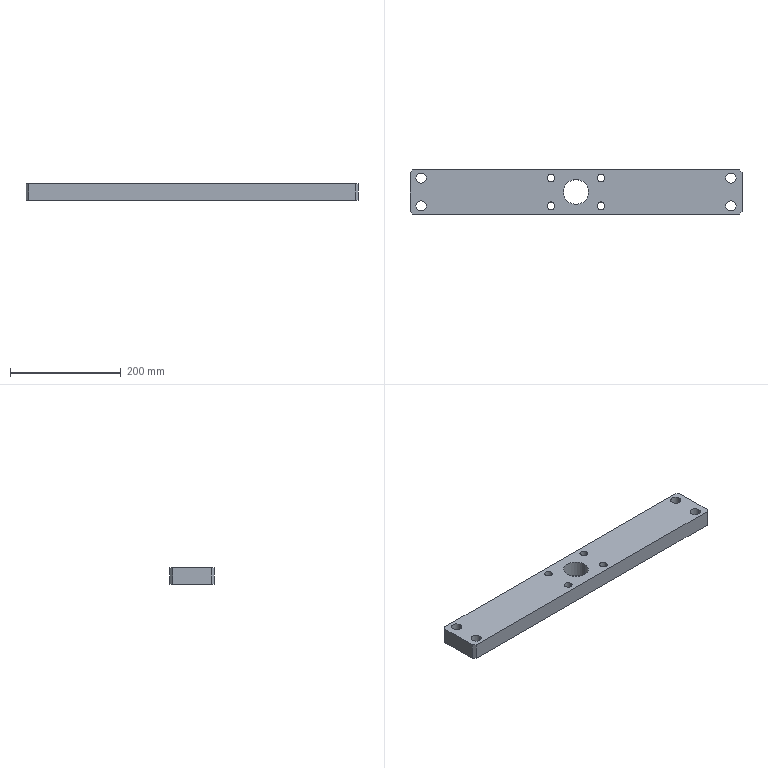Component | SolidWorks | YC1-250-03-01SliderAssembly-1_YC1-250-03-23HydraulicCylinderPressurePlate-1 | 1 solid | 28 faces | box 600 x 80 x 30 mm | volume 1340058 mm3 | cylinder 18 | plane 10 | commonest cylinder face diameters 18.5 x8 14 x8 45 x2 | material Plain Carbon Steel
STEP:
#1=COLOUR_RGB('',0.7922,0.8196,0.9333);
#2=FILL_AREA_STYLE_COLOUR('',#1);
#3=FILL_AREA_STYLE('',(#2));
#4=SURFACE_STYLE_FILL_AREA(#3);
#5=SURFACE_SIDE_STYLE('',(#4));
#6=SURFACE_STYLE_USAGE(.BOTH.,#5);
#7=PRESENTATION_STYLE_ASSIGNMENT((#6));
#8=CARTESIAN_POINT('',(11.388,79.214,-8.465));
#9=VERTEX_POINT('',#8);
#10=CARTESIAN_POINT('',(10.659,79.214,-8.465));
#11=VERTEX_POINT('',#10);
#12=CARTESIAN_POINT('',(11.024,79.214,-8.465));
#13=DIRECTION('',(0.,0.,-1.));
#14=DIRECTION('',(-1.,0.,0.));
#15=AXIS2_PLACEMENT_3D('',#12,#13,#14);
#16=CIRCLE('',#15,0.3642);
#17=EDGE_CURVE('',#9,#11,#16,.T.);
#18=ORIENTED_EDGE('',*,*,#17,.F.);
#19=CARTESIAN_POINT('',(11.388,79.214,-9.646));
#20=VERTEX_POINT('',#19);
#21=CARTESIAN_POINT('',(11.388,79.214,-9.646));
#22=DIRECTION('',(0.,0.,-1.));
#23=VECTOR('',#22,39.37);
#24=LINE('',#21,#23);
#25=EDGE_CURVE('',#9,#20,#24,.T.);
#26=ORIENTED_EDGE('',*,*,#25,.T.);
#27=CARTESIAN_POINT('',(10.659,79.214,-9.646));
#28=VERTEX_POINT('',#27);
#29=CARTESIAN_POINT('',(11.024,79.214,-9.646));
#30=DIRECTION('',(0.,0.,-1.));
#31=DIRECTION('',(-1.,0.,0.));
#32=AXIS2_PLACEMENT_3D('',#29,#30,#31);
#33=CIRCLE('',#32,0.3642);
#34=EDGE_CURVE('',#20,#28,#33,.T.);
#35=ORIENTED_EDGE('',*,*,#34,.T.);
#36=CARTESIAN_POINT('',(10.659,79.214,-9.646));
#37=DIRECTION('',(0.,0.,-1.));
#38=VECTOR('',#37,39.37);
#39=LINE('',#36,#38);
#40=EDGE_CURVE('',#11,#28,#39,.T.);
#41=ORIENTED_EDGE('',*,*,#40,.F.);
#42=EDGE_LOOP('',(#18,#26,#35,#41));
#43=FACE_OUTER_BOUND('',#42,.T.);
#44=CARTESIAN_POINT('',(11.024,79.214,-9.646));
#45=DIRECTION('',(0.,0.,-1.));
#46=DIRECTION('',(-1.,0.,0.));
#47=AXIS2_PLACEMENT_3D('',#44,#45,#46);
#48=CYLINDRICAL_SURFACE('',#47,0.3642);
#49=ADVANCED_FACE('',(#43),#48,.F.);
#50=CARTESIAN_POINT('',(11.388,77.246,-8.465));
#51=VERTEX_POINT('',#50);
#52=CARTESIAN_POINT('',(10.659,77.246,-8.465));
#53=VERTEX_POINT('',#52);
#54=CARTESIAN_POINT('',(11.024,77.246,-8.465));
#55=DIRECTION('',(0.,0.,-1.));
#56=DIRECTION('',(-1.,0.,0.));
#57=AXIS2_PLACEMENT_3D('',#54,#55,#56);
#58=CIRCLE('',#57,0.3642);
#59=EDGE_CURVE('',#51,#53,#58,.T.);
#60=ORIENTED_EDGE('',*,*,#59,.F.);
#61=CARTESIAN_POINT('',(11.388,77.246,-9.646));
#62=VERTEX_POINT('',#61);
#63=CARTESIAN_POINT('',(11.388,77.246,-9.646));
#64=DIRECTION('',(0.,0.,-1.));
#65=VECTOR('',#64,39.37);
#66=LINE('',#63,#65);
#67=EDGE_CURVE('',#51,#62,#66,.T.);
#68=ORIENTED_EDGE('',*,*,#67,.T.);
#69=CARTESIAN_POINT('',(10.659,77.246,-9.646));
#70=VERTEX_POINT('',#69);
#71=CARTESIAN_POINT('',(11.024,77.246,-9.646));
#72=DIRECTION('',(0.,0.,-1.));
#73=DIRECTION('',(-1.,0.,0.));
#74=AXIS2_PLACEMENT_3D('',#71,#72,#73);
#75=CIRCLE('',#74,0.3642);
#76=EDGE_CURVE('',#62,#70,#75,.T.);
#77=ORIENTED_EDGE('',*,*,#76,.T.);
#78=CARTESIAN_POINT('',(10.659,77.246,-9.646));
#79=DIRECTION('',(0.,0.,-1.));
#80=VECTOR('',#79,39.37);
#81=LINE('',#78,#80);
#82=EDGE_CURVE('',#53,#70,#81,.T.);
#83=ORIENTED_EDGE('',*,*,#82,.F.);
#84=EDGE_LOOP('',(#60,#68,#77,#83));
#85=FACE_OUTER_BOUND('',#84,.T.);
#86=CARTESIAN_POINT('',(11.024,77.246,-9.646));
#87=DIRECTION('',(0.,0.,-1.));
#88=DIRECTION('',(-1.,0.,0.));
#89=AXIS2_PLACEMENT_3D('',#86,#87,#88);
#90=CYLINDRICAL_SURFACE('',#89,0.3642);
#91=ADVANCED_FACE('',(#85),#90,.F.);
#92=CARTESIAN_POINT('',(-10.659,77.246,-8.465));
#93=VERTEX_POINT('',#92);
#94=CARTESIAN_POINT('',(-11.388,77.246,-8.465));
#95=VERTEX_POINT('',#94);
#96=CARTESIAN_POINT('',(-11.024,77.246,-8.465));
#97=DIRECTION('',(0.,0.,-1.));
#98=DIRECTION('',(-1.,0.,0.));
#99=AXIS2_PLACEMENT_3D('',#96,#97,#98);
#100=CIRCLE('',#99,0.3642);
#101=EDGE_CURVE('',#93,#95,#100,.T.);
#102=ORIENTED_EDGE('',*,*,#101,.F.);
#103=CARTESIAN_POINT('',(-10.659,77.246,-9.646));
#104=VERTEX_POINT('',#103);
#105=CARTESIAN_POINT('',(-10.659,77.246,-9.646));
#106=DIRECTION('',(0.,0.,-1.));
#107=VECTOR('',#106,39.37);
#108=LINE('',#105,#107);
#109=EDGE_CURVE('',#93,#104,#108,.T.);
#110=ORIENTED_EDGE('',*,*,#109,.T.);
#111=CARTESIAN_POINT('',(-11.388,77.246,-9.646));
#112=VERTEX_POINT('',#111);
#113=CARTESIAN_POINT('',(-11.024,77.246,-9.646));
#114=DIRECTION('',(0.,0.,-1.));
#115=DIRECTION('',(-1.,0.,0.));
#116=AXIS2_PLACEMENT_3D('',#113,#114,#115);
#117=CIRCLE('',#116,0.3642);
#118=EDGE_CURVE('',#104,#112,#117,.T.);
#119=ORIENTED_EDGE('',*,*,#118,.T.);
#120=CARTESIAN_POINT('',(-11.388,77.246,-9.646));
#121=DIRECTION('',(0.,0.,-1.));
#122=VECTOR('',#121,39.37);
#123=LINE('',#120,#122);
#124=EDGE_CURVE('',#95,#112,#123,.T.);
#125=ORIENTED_EDGE('',*,*,#124,.F.);
#126=EDGE_LOOP('',(#102,#110,#119,#125));
#127=FACE_OUTER_BOUND('',#126,.T.);
#128=CARTESIAN_POINT('',(-11.024,77.246,-9.646));
#129=DIRECTION('',(0.,0.,-1.));
#130=DIRECTION('',(-1.,0.,0.));
#131=AXIS2_PLACEMENT_3D('',#128,#129,#130);
#132=CYLINDRICAL_SURFACE('',#131,0.3642);
#133=ADVANCED_FACE('',(#127),#132,.F.);
#134=CARTESIAN_POINT('',(-10.659,79.214,-8.465));
#135=VERTEX_POINT('',#134);
#136=CARTESIAN_POINT('',(-11.388,79.214,-8.465));
#137=VERTEX_POINT('',#136);
#138=CARTESIAN_POINT('',(-11.024,79.214,-8.465));
#139=DIRECTION('',(0.,0.,-1.));
#140=DIRECTION('',(-1.,0.,0.));
#141=AXIS2_PLACEMENT_3D('',#138,#139,#140);
#142=CIRCLE('',#141,0.3642);
#143=EDGE_CURVE('',#135,#137,#142,.T.);
#144=ORIENTED_EDGE('',*,*,#143,.F.);
#145=CARTESIAN_POINT('',(-10.659,79.214,-9.646));
#146=VERTEX_POINT('',#145);
#147=CARTESIAN_POINT('',(-10.659,79.214,-9.646));
#148=DIRECTION('',(0.,0.,-1.));
#149=VECTOR('',#148,39.37);
#150=LINE('',#147,#149);
#151=EDGE_CURVE('',#135,#146,#150,.T.);
#152=ORIENTED_EDGE('',*,*,#151,.T.);
#153=CARTESIAN_POINT('',(-11.388,79.214,-9.646));
#154=VERTEX_POINT('',#153);
#155=CARTESIAN_POINT('',(-11.024,79.214,-9.646));
#156=DIRECTION('',(0.,0.,-1.));
#157=DIRECTION('',(-1.,0.,0.));
#158=AXIS2_PLACEMENT_3D('',#155,#156,#157);
#159=CIRCLE('',#158,0.3642);
#160=EDGE_CURVE('',#146,#154,#159,.T.);
#161=ORIENTED_EDGE('',*,*,#160,.T.);
#162=CARTESIAN_POINT('',(-11.388,79.214,-9.646));
#163=DIRECTION('',(0.,0.,-1.));
#164=VECTOR('',#163,39.37);
#165=LINE('',#162,#164);
#166=EDGE_CURVE('',#137,#154,#165,.T.);
#167=ORIENTED_EDGE('',*,*,#166,.F.);
#168=EDGE_LOOP('',(#144,#152,#161,#167));
#169=FACE_OUTER_BOUND('',#168,.T.);
#170=CARTESIAN_POINT('',(-11.024,79.214,-9.646));
#171=DIRECTION('',(0.,0.,-1.));
#172=DIRECTION('',(-1.,0.,0.));
#173=AXIS2_PLACEMENT_3D('',#170,#171,#172);
#174=CYLINDRICAL_SURFACE('',#173,0.3642);
#175=ADVANCED_FACE('',(#169),#174,.F.);
#176=CARTESIAN_POINT('',(0.8858,78.23,-8.465));
#177=VERTEX_POINT('',#176);
#178=CARTESIAN_POINT('',(-0.8858,78.23,-8.465));
#179=VERTEX_POINT('',#178);
#180=CARTESIAN_POINT('',(0.,78.23,-8.465));
#181=DIRECTION('',(0.,0.,-1.));
#182=DIRECTION('',(-1.,0.,0.));
#183=AXIS2_PLACEMENT_3D('',#180,#181,#182);
#184=CIRCLE('',#183,0.8858);
#185=EDGE_CURVE('',#177,#179,#184,.T.);
#186=ORIENTED_EDGE('',*,*,#185,.F.);
#187=CARTESIAN_POINT('',(0.8858,78.23,-9.646));
#188=VERTEX_POINT('',#187);
#189=CARTESIAN_POINT('',(0.8858,78.23,-9.646));
#190=DIRECTION('',(0.,0.,-1.));
#191=VECTOR('',#190,39.37);
#192=LINE('',#189,#191);
#193=EDGE_CURVE('',#177,#188,#192,.T.);
#194=ORIENTED_EDGE('',*,*,#193,.T.);
#195=CARTESIAN_POINT('',(-0.8858,78.23,-9.646));
#196=VERTEX_POINT('',#195);
#197=CARTESIAN_POINT('',(0.,78.23,-9.646));
#198=DIRECTION('',(0.,0.,-1.));
#199=DIRECTION('',(-1.,0.,0.));
#200=AXIS2_PLACEMENT_3D('',#197,#198,#199);
#201=CIRCLE('',#200,0.8858);
#202=EDGE_CURVE('',#188,#196,#201,.T.);
#203=ORIENTED_EDGE('',*,*,#202,.T.);
#204=CARTESIAN_POINT('',(-0.8858,78.23,-9.646));
#205=DIRECTION('',(0.,0.,-1.));
#206=VECTOR('',#205,39.37);
#207=LINE('',#204,#206);
#208=EDGE_CURVE('',#179,#196,#207,.T.);
#209=ORIENTED_EDGE('',*,*,#208,.F.);
#210=EDGE_LOOP('',(#186,#194,#203,#209));
#211=FACE_OUTER_BOUND('',#210,.T.);
#212=CARTESIAN_POINT('',(0.,78.23,-9.646));
#213=DIRECTION('',(0.,0.,-1.));
#214=DIRECTION('',(-1.,0.,0.));
#215=AXIS2_PLACEMENT_3D('',#212,#213,#214);
#216=CYLINDRICAL_SURFACE('',#215,0.8858);
#217=ADVANCED_FACE('',(#211),#216,.F.);
#218=CARTESIAN_POINT('',(-1.496,77.246,-8.465));
#219=VERTEX_POINT('',#218);
#220=CARTESIAN_POINT('',(-2.047,77.246,-8.465));
#221=VERTEX_POINT('',#220);
#222=CARTESIAN_POINT('',(-1.772,77.246,-8.465));
#223=DIRECTION('',(0.,0.,-1.));
#224=DIRECTION('',(-1.,0.,0.));
#225=AXIS2_PLACEMENT_3D('',#222,#223,#224);
#226=CIRCLE('',#225,0.2756);
#227=EDGE_CURVE('',#219,#221,#226,.T.);
#228=ORIENTED_EDGE('',*,*,#227,.F.);
#229=CARTESIAN_POINT('',(-1.496,77.246,-9.646));
#230=VERTEX_POINT('',#229);
#231=CARTESIAN_POINT('',(-1.496,77.246,-9.646));
#232=DIRECTION('',(0.,0.,-1.));
#233=VECTOR('',#232,39.37);
#234=LINE('',#231,#233);
#235=EDGE_CURVE('',#219,#230,#234,.T.);
#236=ORIENTED_EDGE('',*,*,#235,.T.);
#237=CARTESIAN_POINT('',(-2.047,77.246,-9.646));
#238=VERTEX_POINT('',#237);
#239=CARTESIAN_POINT('',(-1.772,77.246,-9.646));
#240=DIRECTION('',(0.,0.,-1.));
#241=DIRECTION('',(-1.,0.,0.));
#242=AXIS2_PLACEMENT_3D('',#239,#240,#241);
#243=CIRCLE('',#242,0.2756);
#244=EDGE_CURVE('',#230,#238,#243,.T.);
#245=ORIENTED_EDGE('',*,*,#244,.T.);
#246=CARTESIAN_POINT('',(-2.047,77.246,-9.646));
#247=DIRECTION('',(0.,0.,-1.));
#248=VECTOR('',#247,39.37);
#249=LINE('',#246,#248);
#250=EDGE_CURVE('',#221,#238,#249,.T.);
#251=ORIENTED_EDGE('',*,*,#250,.F.);
#252=EDGE_LOOP('',(#228,#236,#245,#251));
#253=FACE_OUTER_BOUND('',#252,.T.);
#254=CARTESIAN_POINT('',(-1.772,77.246,-9.646));
#255=DIRECTION('',(0.,0.,-1.));
#256=DIRECTION('',(-1.,0.,0.));
#257=AXIS2_PLACEMENT_3D('',#254,#255,#256);
#258=CYLINDRICAL_SURFACE('',#257,0.2756);
#259=ADVANCED_FACE('',(#253),#258,.F.);
#260=CARTESIAN_POINT('',(2.047,77.246,-8.465));
#261=VERTEX_POINT('',#260);
#262=CARTESIAN_POINT('',(1.496,77.246,-8.465));
#263=VERTEX_POINT('',#262);
#264=CARTESIAN_POINT('',(1.772,77.246,-8.465));
#265=DIRECTION('',(0.,0.,-1.));
#266=DIRECTION('',(-1.,0.,0.));
#267=AXIS2_PLACEMENT_3D('',#264,#265,#266);
#268=CIRCLE('',#267,0.2756);
#269=EDGE_CURVE('',#261,#263,#268,.T.);
#270=ORIENTED_EDGE('',*,*,#269,.F.);
#271=CARTESIAN_POINT('',(2.047,77.246,-9.646));
#272=VERTEX_POINT('',#271);
#273=CARTESIAN_POINT('',(2.047,77.246,-9.646));
#274=DIRECTION('',(0.,0.,-1.));
#275=VECTOR('',#274,39.37);
#276=LINE('',#273,#275);
#277=EDGE_CURVE('',#261,#272,#276,.T.);
#278=ORIENTED_EDGE('',*,*,#277,.T.);
#279=CARTESIAN_POINT('',(1.496,77.246,-9.646));
#280=VERTEX_POINT('',#279);
#281=CARTESIAN_POINT('',(1.772,77.246,-9.646));
#282=DIRECTION('',(0.,0.,-1.));
#283=DIRECTION('',(-1.,0.,0.));
#284=AXIS2_PLACEMENT_3D('',#281,#282,#283);
#285=CIRCLE('',#284,0.2756);
#286=EDGE_CURVE('',#272,#280,#285,.T.);
#287=ORIENTED_EDGE('',*,*,#286,.T.);
#288=CARTESIAN_POINT('',(1.496,77.246,-9.646));
#289=DIRECTION('',(0.,0.,-1.));
#290=VECTOR('',#289,39.37);
#291=LINE('',#288,#290);
#292=EDGE_CURVE('',#263,#280,#291,.T.);
#293=ORIENTED_EDGE('',*,*,#292,.F.);
#294=EDGE_LOOP('',(#270,#278,#287,#293));
#295=FACE_OUTER_BOUND('',#294,.T.);
#296=CARTESIAN_POINT('',(1.772,77.246,-9.646));
#297=DIRECTION('',(0.,0.,-1.));
#298=DIRECTION('',(-1.,0.,0.));
#299=AXIS2_PLACEMENT_3D('',#296,#297,#298);
#300=CYLINDRICAL_SURFACE('',#299,0.2756);
#301=ADVANCED_FACE('',(#295),#300,.F.);
#302=CARTESIAN_POINT('',(2.047,79.214,-8.465));
#303=VERTEX_POINT('',#302);
#304=CARTESIAN_POINT('',(1.496,79.214,-8.465));
#305=VERTEX_POINT('',#304);
#306=CARTESIAN_POINT('',(1.772,79.214,-8.465));
#307=DIRECTION('',(0.,0.,-1.));
#308=DIRECTION('',(-1.,0.,0.));
#309=AXIS2_PLACEMENT_3D('',#306,#307,#308);
#310=CIRCLE('',#309,0.2756);
#311=EDGE_CURVE('',#303,#305,#310,.T.);
#312=ORIENTED_EDGE('',*,*,#311,.F.);
#313=CARTESIAN_POINT('',(2.047,79.214,-9.646));
#314=VERTEX_POINT('',#313);
#315=CARTESIAN_POINT('',(2.047,79.214,-9.646));
#316=DIRECTION('',(0.,0.,-1.));
#317=VECTOR('',#316,39.37);
#318=LINE('',#315,#317);
#319=EDGE_CURVE('',#303,#314,#318,.T.);
#320=ORIENTED_EDGE('',*,*,#319,.T.);
#321=CARTESIAN_POINT('',(1.496,79.214,-9.646));
#322=VERTEX_POINT('',#321);
#323=CARTESIAN_POINT('',(1.772,79.214,-9.646));
#324=DIRECTION('',(0.,0.,-1.));
#325=DIRECTION('',(-1.,0.,0.));
#326=AXIS2_PLACEMENT_3D('',#323,#324,#325);
#327=CIRCLE('',#326,0.2756);
#328=EDGE_CURVE('',#314,#322,#327,.T.);
#329=ORIENTED_EDGE('',*,*,#328,.T.);
#330=CARTESIAN_POINT('',(1.496,79.214,-9.646));
#331=DIRECTION('',(0.,0.,-1.));
#332=VECTOR('',#331,39.37);
#333=LINE('',#330,#332);
#334=EDGE_CURVE('',#305,#322,#333,.T.);
#335=ORIENTED_EDGE('',*,*,#334,.F.);
#336=EDGE_LOOP('',(#312,#320,#329,#335));
#337=FACE_OUTER_BOUND('',#336,.T.);
#338=CARTESIAN_POINT('',(1.772,79.214,-9.646));
#339=DIRECTION('',(0.,0.,-1.));
#340=DIRECTION('',(-1.,0.,0.));
#341=AXIS2_PLACEMENT_3D('',#338,#339,#340);
#342=CYLINDRICAL_SURFACE('',#341,0.2756);
#343=ADVANCED_FACE('',(#337),#342,.F.);
#344=CARTESIAN_POINT('',(-1.496,79.214,-8.465));
#345=VERTEX_POINT('',#344);
#346=CARTESIAN_POINT('',(-2.047,79.214,-8.465));
#347=VERTEX_POINT('',#346);
#348=CARTESIAN_POINT('',(-1.772,79.214,-8.465));
#349=DIRECTION('',(0.,0.,-1.));
#350=DIRECTION('',(-1.,0.,0.));
#351=AXIS2_PLACEMENT_3D('',#348,#349,#350);
#352=CIRCLE('',#351,0.2756);
#353=EDGE_CURVE('',#345,#347,#352,.T.);
#354=ORIENTED_EDGE('',*,*,#353,.F.);
#355=CARTESIAN_POINT('',(-1.496,79.214,-9.646));
#356=VERTEX_POINT('',#355);
#357=CARTESIAN_POINT('',(-1.496,79.214,-9.646));
#358=DIRECTION('',(0.,0.,-1.));
#359=VECTOR('',#358,39.37);
#360=LINE('',#357,#359);
#361=EDGE_CURVE('',#345,#356,#360,.T.);
#362=ORIENTED_EDGE('',*,*,#361,.T.);
#363=CARTESIAN_POINT('',(-2.047,79.214,-9.646));
#364=VERTEX_POINT('',#363);
#365=CARTESIAN_POINT('',(-1.772,79.214,-9.646));
#366=DIRECTION('',(0.,0.,-1.));
#367=DIRECTION('',(-1.,0.,0.));
#368=AXIS2_PLACEMENT_3D('',#365,#366,#367);
#369=CIRCLE('',#368,0.2756);
#370=EDGE_CURVE('',#356,#364,#369,.T.);
#371=ORIENTED_EDGE('',*,*,#370,.T.);
#372=CARTESIAN_POINT('',(-2.047,79.214,-9.646));
#373=DIRECTION('',(0.,0.,-1.));
#374=VECTOR('',#373,39.37);
#375=LINE('',#372,#374);
#376=EDGE_CURVE('',#347,#364,#375,.T.);
#377=ORIENTED_EDGE('',*,*,#376,.F.);
#378=EDGE_LOOP('',(#354,#362,#371,#377));
#379=FACE_OUTER_BOUND('',#378,.T.);
#380=CARTESIAN_POINT('',(-1.772,79.214,-9.646));
#381=DIRECTION('',(0.,0.,-1.));
#382=DIRECTION('',(-1.,0.,0.));
#383=AXIS2_PLACEMENT_3D('',#380,#381,#382);
#384=CYLINDRICAL_SURFACE('',#383,0.2756);
#385=ADVANCED_FACE('',(#379),#384,.F.);
#386=CARTESIAN_POINT('',(11.614,76.655,-9.646));
#387=VERTEX_POINT('',#386);
#388=CARTESIAN_POINT('',(11.811,76.852,-9.646));
#389=VERTEX_POINT('',#388);
#390=CARTESIAN_POINT('',(11.614,76.655,-9.646));
#391=DIRECTION('',(0.7071,0.7071,0.));
#392=VECTOR('',#391,39.37);
#393=LINE('',#390,#392);
#394=EDGE_CURVE('',#387,#389,#393,.T.);
#395=ORIENTED_EDGE('',*,*,#394,.F.);
#396=CARTESIAN_POINT('',(-11.614,76.655,-9.646));
#397=VERTEX_POINT('',#396);
#398=CARTESIAN_POINT('',(-11.811,76.655,-9.646));
#399=DIRECTION('',(1.,0.,0.));
#400=VECTOR('',#399,39.37);
#401=LINE('',#398,#400);
#402=EDGE_CURVE('',#397,#387,#401,.T.);
#403=ORIENTED_EDGE('',*,*,#402,.F.);
#404=CARTESIAN_POINT('',(-11.811,76.852,-9.646));
#405=VERTEX_POINT('',#404);
#406=CARTESIAN_POINT('',(-11.811,76.852,-9.646));
#407=DIRECTION('',(0.7071,-0.7071,0.));
#408=VECTOR('',#407,39.37);
#409=LINE('',#406,#408);
#410=EDGE_CURVE('',#405,#397,#409,.T.);
#411=ORIENTED_EDGE('',*,*,#410,.F.);
#412=CARTESIAN_POINT('',(-11.811,79.608,-9.646));
#413=VERTEX_POINT('',#412);
#414=CARTESIAN_POINT('',(-11.811,76.655,-9.646));
#415=DIRECTION('',(0.,-1.,0.));
#416=VECTOR('',#415,39.37);
#417=LINE('',#414,#416);
#418=EDGE_CURVE('',#413,#405,#417,.T.);
#419=ORIENTED_EDGE('',*,*,#418,.F.);
#420=CARTESIAN_POINT('',(-11.614,79.805,-9.646));
#421=VERTEX_POINT('',#420);
#422=CARTESIAN_POINT('',(-11.614,79.805,-9.646));
#423=DIRECTION('',(-0.7071,-0.7071,0.));
#424=VECTOR('',#423,39.37);
#425=LINE('',#422,#424);
#426=EDGE_CURVE('',#421,#413,#425,.T.);
#427=ORIENTED_EDGE('',*,*,#426,.F.);
#428=CARTESIAN_POINT('',(11.614,79.805,-9.646));
#429=VERTEX_POINT('',#428);
#430=CARTESIAN_POINT('',(-11.811,79.805,-9.646));
#431=DIRECTION('',(-1.,0.,0.));
#432=VECTOR('',#431,39.37);
#433=LINE('',#430,#432);
#434=EDGE_CURVE('',#429,#421,#433,.T.);
#435=ORIENTED_EDGE('',*,*,#434,.F.);
#436=CARTESIAN_POINT('',(11.811,79.608,-9.646));
#437=VERTEX_POINT('',#436);
#438=CARTESIAN_POINT('',(11.811,79.608,-9.646));
#439=DIRECTION('',(-0.7071,0.7071,0.));
#440=VECTOR('',#439,39.37);
#441=LINE('',#438,#440);
#442=EDGE_CURVE('',#437,#429,#441,.T.);
#443=ORIENTED_EDGE('',*,*,#442,.F.);
#444=CARTESIAN_POINT('',(11.811,76.655,-9.646));
#445=DIRECTION('',(0.,1.,0.));
#446=VECTOR('',#445,39.37);
#447=LINE('',#444,#446);
#448=EDGE_CURVE('',#389,#437,#447,.T.);
#449=ORIENTED_EDGE('',*,*,#448,.F.);
#450=EDGE_LOOP('',(#395,#403,#411,#419,#427,#435,#443,#449));
#451=FACE_OUTER_BOUND('',#450,.T.);
#452=CARTESIAN_POINT('',(11.024,79.214,-9.646));
#453=DIRECTION('',(0.,0.,-1.));
#454=DIRECTION('',(-1.,0.,0.));
#455=AXIS2_PLACEMENT_3D('',#452,#453,#454);
#456=CIRCLE('',#455,0.3642);
#457=EDGE_CURVE('',#28,#20,#456,.T.);
#458=ORIENTED_EDGE('',*,*,#457,.F.);
#459=ORIENTED_EDGE('',*,*,#34,.F.);
#460=EDGE_LOOP('',(#458,#459));
#461=FACE_BOUND('',#460,.T.);
#462=CARTESIAN_POINT('',(11.024,77.246,-9.646));
#463=DIRECTION('',(0.,0.,-1.));
#464=DIRECTION('',(-1.,0.,0.));
#465=AXIS2_PLACEMENT_3D('',#462,#463,#464);
#466=CIRCLE('',#465,0.3642);
#467=EDGE_CURVE('',#70,#62,#466,.T.);
#468=ORIENTED_EDGE('',*,*,#467,.F.);
#469=ORIENTED_EDGE('',*,*,#76,.F.);
#470=EDGE_LOOP('',(#468,#469));
#471=FACE_BOUND('',#470,.T.);
#472=CARTESIAN_POINT('',(-11.024,77.246,-9.646));
#473=DIRECTION('',(0.,0.,-1.));
#474=DIRECTION('',(-1.,0.,0.));
#475=AXIS2_PLACEMENT_3D('',#472,#473,#474);
#476=CIRCLE('',#475,0.3642);
#477=EDGE_CURVE('',#112,#104,#476,.T.);
#478=ORIENTED_EDGE('',*,*,#477,.F.);
#479=ORIENTED_EDGE('',*,*,#118,.F.);
#480=EDGE_LOOP('',(#478,#479));
#481=FACE_BOUND('',#480,.T.);
#482=CARTESIAN_POINT('',(-11.024,79.214,-9.646));
#483=DIRECTION('',(0.,0.,-1.));
#484=DIRECTION('',(-1.,0.,0.));
#485=AXIS2_PLACEMENT_3D('',#482,#483,#484);
#486=CIRCLE('',#485,0.3642);
#487=EDGE_CURVE('',#154,#146,#486,.T.);
#488=ORIENTED_EDGE('',*,*,#487,.F.);
#489=ORIENTED_EDGE('',*,*,#160,.F.);
#490=EDGE_LOOP('',(#488,#489));
#491=FACE_BOUND('',#490,.T.);
#492=CARTESIAN_POINT('',(0.,78.23,-9.646));
#493=DIRECTION('',(0.,0.,-1.));
#494=DIRECTION('',(-1.,0.,0.));
#495=AXIS2_PLACEMENT_3D('',#492,#493,#494);
#496=CIRCLE('',#495,0.8858);
#497=EDGE_CURVE('',#196,#188,#496,.T.);
#498=ORIENTED_EDGE('',*,*,#497,.F.);
#499=ORIENTED_EDGE('',*,*,#202,.F.);
#500=EDGE_LOOP('',(#498,#499));
#501=FACE_BOUND('',#500,.T.);
#502=CARTESIAN_POINT('',(-1.772,77.246,-9.646));
#503=DIRECTION('',(0.,0.,-1.));
#504=DIRECTION('',(-1.,0.,0.));
#505=AXIS2_PLACEMENT_3D('',#502,#503,#504);
#506=CIRCLE('',#505,0.2756);
#507=EDGE_CURVE('',#238,#230,#506,.T.);
#508=ORIENTED_EDGE('',*,*,#507,.F.);
#509=ORIENTED_EDGE('',*,*,#244,.F.);
#510=EDGE_LOOP('',(#508,#509));
#511=FACE_BOUND('',#510,.T.);
#512=CARTESIAN_POINT('',(1.772,77.246,-9.646));
#513=DIRECTION('',(0.,0.,-1.));
#514=DIRECTION('',(-1.,0.,0.));
#515=AXIS2_PLACEMENT_3D('',#512,#513,#514);
#516=CIRCLE('',#515,0.2756);
#517=EDGE_CURVE('',#280,#272,#516,.T.);
#518=ORIENTED_EDGE('',*,*,#517,.F.);
#519=ORIENTED_EDGE('',*,*,#286,.F.);
#520=EDGE_LOOP('',(#518,#519));
#521=FACE_BOUND('',#520,.T.);
#522=CARTESIAN_POINT('',(1.772,79.214,-9.646));
#523=DIRECTION('',(0.,0.,-1.));
#524=DIRECTION('',(-1.,0.,0.));
#525=AXIS2_PLACEMENT_3D('',#522,#523,#524);
#526=CIRCLE('',#525,0.2756);
#527=EDGE_CURVE('',#322,#314,#526,.T.);
#528=ORIENTED_EDGE('',*,*,#527,.F.);
#529=ORIENTED_EDGE('',*,*,#328,.F.);
#530=EDGE_LOOP('',(#528,#529));
#531=FACE_BOUND('',#530,.T.);
#532=CARTESIAN_POINT('',(-1.772,79.214,-9.646));
#533=DIRECTION('',(0.,0.,-1.));
#534=DIRECTION('',(-1.,0.,0.));
#535=AXIS2_PLACEMENT_3D('',#532,#533,#534);
#536=CIRCLE('',#535,0.2756);
#537=EDGE_CURVE('',#364,#356,#536,.T.);
#538=ORIENTED_EDGE('',*,*,#537,.F.);
#539=ORIENTED_EDGE('',*,*,#370,.F.);
#540=EDGE_LOOP('',(#538,#539));
#541=FACE_BOUND('',#540,.T.);
#542=CARTESIAN_POINT('',(-11.811,76.655,-9.646));
#543=DIRECTION('',(0.,0.,1.));
#544=DIRECTION('',(1.,0.,0.));
#545=AXIS2_PLACEMENT_3D('',#542,#543,#544);
#546=PLANE('',#545);
#547=ADVANCED_FACE('',(#451,#461,#471,#481,#491,#501,#511,#521,#531,#541),#546,.F.);
#548=CARTESIAN_POINT('',(11.811,76.852,-8.465));
#549=VERTEX_POINT('',#548);
#550=CARTESIAN_POINT('',(11.811,76.852,-8.465));
#551=DIRECTION('',(0.,0.,1.));
#552=VECTOR('',#551,39.37);
#553=LINE('',#550,#552);
#554=EDGE_CURVE('',#389,#549,#553,.T.);
#555=ORIENTED_EDGE('',*,*,#554,.F.);
#556=ORIENTED_EDGE('',*,*,#448,.T.);
#557=CARTESIAN_POINT('',(11.811,79.608,-8.465));
#558=VERTEX_POINT('',#557);
#559=CARTESIAN_POINT('',(11.811,79.608,-8.465));
#560=DIRECTION('',(0.,0.,-1.));
#561=VECTOR('',#560,39.37);
#562=LINE('',#559,#561);
#563=EDGE_CURVE('',#558,#437,#562,.T.);
#564=ORIENTED_EDGE('',*,*,#563,.F.);
#565=CARTESIAN_POINT('',(11.811,79.805,-8.465));
#566=DIRECTION('',(0.,1.,0.));
#567=VECTOR('',#566,39.37);
#568=LINE('',#565,#567);
#569=EDGE_CURVE('',#549,#558,#568,.T.);
#570=ORIENTED_EDGE('',*,*,#569,.F.);
#571=EDGE_LOOP('',(#555,#556,#564,#570));
#572=FACE_OUTER_BOUND('',#571,.T.);
#573=CARTESIAN_POINT('',(11.811,79.805,-8.465));
#574=DIRECTION('',(-1.,0.,0.));
#575=DIRECTION('',(0.,0.,1.));
#576=AXIS2_PLACEMENT_3D('',#573,#574,#575);
#577=PLANE('',#576);
#578=ADVANCED_FACE('',(#572),#577,.F.);
#579=CARTESIAN_POINT('',(11.614,76.655,-8.465));
#580=VERTEX_POINT('',#579);
#581=CARTESIAN_POINT('',(11.614,76.655,-8.465));
#582=DIRECTION('',(0.,0.,1.));
#583=VECTOR('',#582,39.37);
#584=LINE('',#581,#583);
#585=EDGE_CURVE('',#387,#580,#584,.T.);
#586=ORIENTED_EDGE('',*,*,#585,.F.);
#587=ORIENTED_EDGE('',*,*,#394,.T.);
#588=ORIENTED_EDGE('',*,*,#554,.T.);
#589=CARTESIAN_POINT('',(11.811,76.852,-8.465));
#590=DIRECTION('',(0.7071,0.7071,0.));
#591=VECTOR('',#590,39.37);
#592=LINE('',#589,#591);
#593=EDGE_CURVE('',#580,#549,#592,.T.);
#594=ORIENTED_EDGE('',*,*,#593,.F.);
#595=EDGE_LOOP('',(#586,#587,#588,#594));
#596=FACE_OUTER_BOUND('',#595,.T.);
#597=CARTESIAN_POINT('',(11.811,76.852,-8.465));
#598=DIRECTION('',(-0.7071,0.7071,0.));
#599=DIRECTION('',(-0.7071,-0.7071,0.));
#600=AXIS2_PLACEMENT_3D('',#597,#598,#599);
#601=PLANE('',#600);
#602=ADVANCED_FACE('',(#596),#601,.F.);
#603=ORIENTED_EDGE('',*,*,#585,.T.);
#604=CARTESIAN_POINT('',(-11.614,76.655,-8.465));
#605=VERTEX_POINT('',#604);
#606=CARTESIAN_POINT('',(-11.811,76.655,-8.465));
#607=DIRECTION('',(1.,0.,0.));
#608=VECTOR('',#607,39.37);
#609=LINE('',#606,#608);
#610=EDGE_CURVE('',#605,#580,#609,.T.);
#611=ORIENTED_EDGE('',*,*,#610,.F.);
#612=CARTESIAN_POINT('',(-11.614,76.655,-8.465));
#613=DIRECTION('',(0.,0.,1.));
#614=VECTOR('',#613,39.37);
#615=LINE('',#612,#614);
#616=EDGE_CURVE('',#397,#605,#615,.T.);
#617=ORIENTED_EDGE('',*,*,#616,.F.);
#618=ORIENTED_EDGE('',*,*,#402,.T.);
#619=EDGE_LOOP('',(#603,#611,#617,#618));
#620=FACE_OUTER_BOUND('',#619,.T.);
#621=CARTESIAN_POINT('',(-11.811,76.655,-8.465));
#622=DIRECTION('',(-0.,1.,0.));
#623=DIRECTION('',(-1.,-0.,0.));
#624=AXIS2_PLACEMENT_3D('',#621,#622,#623);
#625=PLANE('',#624);
#626=ADVANCED_FACE('',(#620),#625,.F.);
#627=CARTESIAN_POINT('',(-11.811,76.852,-8.465));
#628=VERTEX_POINT('',#627);
#629=CARTESIAN_POINT('',(-11.811,76.852,-8.465));
#630=DIRECTION('',(0.,0.,1.));
#631=VECTOR('',#630,39.37);
#632=LINE('',#629,#631);
#633=EDGE_CURVE('',#405,#628,#632,.T.);
#634=ORIENTED_EDGE('',*,*,#633,.F.);
#635=ORIENTED_EDGE('',*,*,#410,.T.);
#636=ORIENTED_EDGE('',*,*,#616,.T.);
#637=CARTESIAN_POINT('',(-11.614,76.655,-8.465));
#638=DIRECTION('',(0.7071,-0.7071,0.));
#639=VECTOR('',#638,39.37);
#640=LINE('',#637,#639);
#641=EDGE_CURVE('',#628,#605,#640,.T.);
#642=ORIENTED_EDGE('',*,*,#641,.F.);
#643=EDGE_LOOP('',(#634,#635,#636,#642));
#644=FACE_OUTER_BOUND('',#643,.T.);
#645=CARTESIAN_POINT('',(-11.614,76.655,-8.465));
#646=DIRECTION('',(0.7071,0.7071,0.));
#647=DIRECTION('',(-0.7071,0.7071,0.));
#648=AXIS2_PLACEMENT_3D('',#645,#646,#647);
#649=PLANE('',#648);
#650=ADVANCED_FACE('',(#644),#649,.F.);
#651=ORIENTED_EDGE('',*,*,#633,.T.);
#652=CARTESIAN_POINT('',(-11.811,79.608,-8.465));
#653=VERTEX_POINT('',#652);
#654=CARTESIAN_POINT('',(-11.811,79.805,-8.465));
#655=DIRECTION('',(0.,-1.,0.));
#656=VECTOR('',#655,39.37);
#657=LINE('',#654,#656);
#658=EDGE_CURVE('',#653,#628,#657,.T.);
#659=ORIENTED_EDGE('',*,*,#658,.F.);
#660=CARTESIAN_POINT('',(-11.811,79.608,-8.465));
#661=DIRECTION('',(0.,0.,1.));
#662=VECTOR('',#661,39.37);
#663=LINE('',#660,#662);
#664=EDGE_CURVE('',#413,#653,#663,.T.);
#665=ORIENTED_EDGE('',*,*,#664,.F.);
#666=ORIENTED_EDGE('',*,*,#418,.T.);
#667=EDGE_LOOP('',(#651,#659,#665,#666));
#668=FACE_OUTER_BOUND('',#667,.T.);
#669=CARTESIAN_POINT('',(-11.811,79.805,-8.465));
#670=DIRECTION('',(1.,0.,0.));
#671=DIRECTION('',(0.,0.,-1.));
#672=AXIS2_PLACEMENT_3D('',#669,#670,#671);
#673=PLANE('',#672);
#674=ADVANCED_FACE('',(#668),#673,.F.);
#675=CARTESIAN_POINT('',(-11.614,79.805,-8.465));
#676=VERTEX_POINT('',#675);
#677=CARTESIAN_POINT('',(-11.614,79.805,-8.465));
#678=DIRECTION('',(0.,0.,1.));
#679=VECTOR('',#678,39.37);
#680=LINE('',#677,#679);
#681=EDGE_CURVE('',#421,#676,#680,.T.);
#682=ORIENTED_EDGE('',*,*,#681,.F.);
#683=ORIENTED_EDGE('',*,*,#426,.T.);
#684=ORIENTED_EDGE('',*,*,#664,.T.);
#685=CARTESIAN_POINT('',(-11.811,79.608,-8.465));
#686=DIRECTION('',(-0.7071,-0.7071,0.));
#687=VECTOR('',#686,39.37);
#688=LINE('',#685,#687);
#689=EDGE_CURVE('',#676,#653,#688,.T.);
#690=ORIENTED_EDGE('',*,*,#689,.F.);
#691=EDGE_LOOP('',(#682,#683,#684,#690));
#692=FACE_OUTER_BOUND('',#691,.T.);
#693=CARTESIAN_POINT('',(-11.811,79.608,-8.465));
#694=DIRECTION('',(0.7071,-0.7071,0.));
#695=DIRECTION('',(0.7071,0.7071,0.));
#696=AXIS2_PLACEMENT_3D('',#693,#694,#695);
#697=PLANE('',#696);
#698=ADVANCED_FACE('',(#692),#697,.F.);
#699=CARTESIAN_POINT('',(11.614,79.805,-8.465));
#700=VERTEX_POINT('',#699);
#701=CARTESIAN_POINT('',(11.614,79.805,-8.465));
#702=DIRECTION('',(0.,0.,1.));
#703=VECTOR('',#702,39.37);
#704=LINE('',#701,#703);
#705=EDGE_CURVE('',#429,#700,#704,.T.);
#706=ORIENTED_EDGE('',*,*,#705,.F.);
#707=ORIENTED_EDGE('',*,*,#434,.T.);
#708=ORIENTED_EDGE('',*,*,#681,.T.);
#709=CARTESIAN_POINT('',(-11.811,79.805,-8.465));
#710=DIRECTION('',(-1.,-0.,0.));
#711=VECTOR('',#710,39.37);
#712=LINE('',#709,#711);
#713=EDGE_CURVE('',#700,#676,#712,.T.);
#714=ORIENTED_EDGE('',*,*,#713,.F.);
#715=EDGE_LOOP('',(#706,#707,#708,#714));
#716=FACE_OUTER_BOUND('',#715,.T.);
#717=CARTESIAN_POINT('',(-11.811,79.805,-8.465));
#718=DIRECTION('',(0.,-1.,0.));
#719=DIRECTION('',(1.,0.,0.));
#720=AXIS2_PLACEMENT_3D('',#717,#718,#719);
#721=PLANE('',#720);
#722=ADVANCED_FACE('',(#716),#721,.F.);
#723=ORIENTED_EDGE('',*,*,#563,.T.);
#724=ORIENTED_EDGE('',*,*,#442,.T.);
#725=ORIENTED_EDGE('',*,*,#705,.T.);
#726=CARTESIAN_POINT('',(11.614,79.805,-8.465));
#727=DIRECTION('',(-0.7071,0.7071,0.));
#728=VECTOR('',#727,39.37);
#729=LINE('',#726,#728);
#730=EDGE_CURVE('',#558,#700,#729,.T.);
#731=ORIENTED_EDGE('',*,*,#730,.F.);
#732=EDGE_LOOP('',(#723,#724,#725,#731));
#733=FACE_OUTER_BOUND('',#732,.T.);
#734=CARTESIAN_POINT('',(11.614,79.805,-8.465));
#735=DIRECTION('',(-0.7071,-0.7071,0.));
#736=DIRECTION('',(0.7071,-0.7071,0.));
#737=AXIS2_PLACEMENT_3D('',#734,#735,#736);
#738=PLANE('',#737);
#739=ADVANCED_FACE('',(#733),#738,.F.);
#740=ORIENTED_EDGE('',*,*,#25,.F.);
#741=CARTESIAN_POINT('',(11.024,79.214,-8.465));
#742=DIRECTION('',(0.,0.,-1.));
#743=DIRECTION('',(-1.,0.,0.));
#744=AXIS2_PLACEMENT_3D('',#741,#742,#743);
#745=CIRCLE('',#744,0.3642);
#746=EDGE_CURVE('',#11,#9,#745,.T.);
#747=ORIENTED_EDGE('',*,*,#746,.F.);
#748=ORIENTED_EDGE('',*,*,#40,.T.);
#749=ORIENTED_EDGE('',*,*,#457,.T.);
#750=EDGE_LOOP('',(#740,#747,#748,#749));
#751=FACE_OUTER_BOUND('',#750,.T.);
#752=CARTESIAN_POINT('',(11.024,79.214,-9.646));
#753=DIRECTION('',(0.,0.,-1.));
#754=DIRECTION('',(-1.,0.,0.));
#755=AXIS2_PLACEMENT_3D('',#752,#753,#754);
#756=CYLINDRICAL_SURFACE('',#755,0.3642);
#757=ADVANCED_FACE('',(#751),#756,.F.);
#758=ORIENTED_EDGE('',*,*,#67,.F.);
#759=CARTESIAN_POINT('',(11.024,77.246,-8.465));
#760=DIRECTION('',(0.,0.,-1.));
#761=DIRECTION('',(-1.,0.,0.));
#762=AXIS2_PLACEMENT_3D('',#759,#760,#761);
#763=CIRCLE('',#762,0.3642);
#764=EDGE_CURVE('',#53,#51,#763,.T.);
#765=ORIENTED_EDGE('',*,*,#764,.F.);
#766=ORIENTED_EDGE('',*,*,#82,.T.);
#767=ORIENTED_EDGE('',*,*,#467,.T.);
#768=EDGE_LOOP('',(#758,#765,#766,#767));
#769=FACE_OUTER_BOUND('',#768,.T.);
#770=CARTESIAN_POINT('',(11.024,77.246,-9.646));
#771=DIRECTION('',(0.,0.,-1.));
#772=DIRECTION('',(-1.,0.,0.));
#773=AXIS2_PLACEMENT_3D('',#770,#771,#772);
#774=CYLINDRICAL_SURFACE('',#773,0.3642);
#775=ADVANCED_FACE('',(#769),#774,.F.);
#776=ORIENTED_EDGE('',*,*,#109,.F.);
#777=CARTESIAN_POINT('',(-11.024,77.246,-8.465));
#778=DIRECTION('',(0.,0.,-1.));
#779=DIRECTION('',(-1.,0.,0.));
#780=AXIS2_PLACEMENT_3D('',#777,#778,#779);
#781=CIRCLE('',#780,0.3642);
#782=EDGE_CURVE('',#95,#93,#781,.T.);
#783=ORIENTED_EDGE('',*,*,#782,.F.);
#784=ORIENTED_EDGE('',*,*,#124,.T.);
#785=ORIENTED_EDGE('',*,*,#477,.T.);
#786=EDGE_LOOP('',(#776,#783,#784,#785));
#787=FACE_OUTER_BOUND('',#786,.T.);
#788=CARTESIAN_POINT('',(-11.024,77.246,-9.646));
#789=DIRECTION('',(0.,0.,-1.));
#790=DIRECTION('',(-1.,0.,0.));
#791=AXIS2_PLACEMENT_3D('',#788,#789,#790);
#792=CYLINDRICAL_SURFACE('',#791,0.3642);
#793=ADVANCED_FACE('',(#787),#792,.F.);
#794=ORIENTED_EDGE('',*,*,#151,.F.);
#795=CARTESIAN_POINT('',(-11.024,79.214,-8.465));
#796=DIRECTION('',(0.,0.,-1.));
#797=DIRECTION('',(-1.,0.,0.));
#798=AXIS2_PLACEMENT_3D('',#795,#796,#797);
#799=CIRCLE('',#798,0.3642);
#800=EDGE_CURVE('',#137,#135,#799,.T.);
#801=ORIENTED_EDGE('',*,*,#800,.F.);
#802=ORIENTED_EDGE('',*,*,#166,.T.);
#803=ORIENTED_EDGE('',*,*,#487,.T.);
#804=EDGE_LOOP('',(#794,#801,#802,#803));
#805=FACE_OUTER_BOUND('',#804,.T.);
#806=CARTESIAN_POINT('',(-11.024,79.214,-9.646));
#807=DIRECTION('',(0.,0.,-1.));
#808=DIRECTION('',(-1.,0.,0.));
#809=AXIS2_PLACEMENT_3D('',#806,#807,#808);
#810=CYLINDRICAL_SURFACE('',#809,0.3642);
#811=ADVANCED_FACE('',(#805),#810,.F.);
#812=ORIENTED_EDGE('',*,*,#193,.F.);
#813=CARTESIAN_POINT('',(0.,78.23,-8.465));
#814=DIRECTION('',(0.,0.,-1.));
#815=DIRECTION('',(-1.,0.,0.));
#816=AXIS2_PLACEMENT_3D('',#813,#814,#815);
#817=CIRCLE('',#816,0.8858);
#818=EDGE_CURVE('',#179,#177,#817,.T.);
#819=ORIENTED_EDGE('',*,*,#818,.F.);
#820=ORIENTED_EDGE('',*,*,#208,.T.);
#821=ORIENTED_EDGE('',*,*,#497,.T.);
#822=EDGE_LOOP('',(#812,#819,#820,#821));
#823=FACE_OUTER_BOUND('',#822,.T.);
#824=CARTESIAN_POINT('',(0.,78.23,-9.646));
#825=DIRECTION('',(0.,0.,-1.));
#826=DIRECTION('',(-1.,0.,0.));
#827=AXIS2_PLACEMENT_3D('',#824,#825,#826);
#828=CYLINDRICAL_SURFACE('',#827,0.8858);
#829=ADVANCED_FACE('',(#823),#828,.F.);
#830=ORIENTED_EDGE('',*,*,#235,.F.);
#831=CARTESIAN_POINT('',(-1.772,77.246,-8.465));
#832=DIRECTION('',(0.,0.,-1.));
#833=DIRECTION('',(-1.,0.,0.));
#834=AXIS2_PLACEMENT_3D('',#831,#832,#833);
#835=CIRCLE('',#834,0.2756);
#836=EDGE_CURVE('',#221,#219,#835,.T.);
#837=ORIENTED_EDGE('',*,*,#836,.F.);
#838=ORIENTED_EDGE('',*,*,#250,.T.);
#839=ORIENTED_EDGE('',*,*,#507,.T.);
#840=EDGE_LOOP('',(#830,#837,#838,#839));
#841=FACE_OUTER_BOUND('',#840,.T.);
#842=CARTESIAN_POINT('',(-1.772,77.246,-9.646));
#843=DIRECTION('',(0.,0.,-1.));
#844=DIRECTION('',(-1.,0.,0.));
#845=AXIS2_PLACEMENT_3D('',#842,#843,#844);
#846=CYLINDRICAL_SURFACE('',#845,0.2756);
#847=ADVANCED_FACE('',(#841),#846,.F.);
#848=ORIENTED_EDGE('',*,*,#277,.F.);
#849=CARTESIAN_POINT('',(1.772,77.246,-8.465));
#850=DIRECTION('',(0.,0.,-1.));
#851=DIRECTION('',(-1.,0.,0.));
#852=AXIS2_PLACEMENT_3D('',#849,#850,#851);
#853=CIRCLE('',#852,0.2756);
#854=EDGE_CURVE('',#263,#261,#853,.T.);
#855=ORIENTED_EDGE('',*,*,#854,.F.);
#856=ORIENTED_EDGE('',*,*,#292,.T.);
#857=ORIENTED_EDGE('',*,*,#517,.T.);
#858=EDGE_LOOP('',(#848,#855,#856,#857));
#859=FACE_OUTER_BOUND('',#858,.T.);
#860=CARTESIAN_POINT('',(1.772,77.246,-9.646));
#861=DIRECTION('',(0.,0.,-1.));
#862=DIRECTION('',(-1.,0.,0.));
#863=AXIS2_PLACEMENT_3D('',#860,#861,#862);
#864=CYLINDRICAL_SURFACE('',#863,0.2756);
#865=ADVANCED_FACE('',(#859),#864,.F.);
#866=ORIENTED_EDGE('',*,*,#319,.F.);
#867=CARTESIAN_POINT('',(1.772,79.214,-8.465));
#868=DIRECTION('',(0.,0.,-1.));
#869=DIRECTION('',(-1.,0.,0.));
#870=AXIS2_PLACEMENT_3D('',#867,#868,#869);
#871=CIRCLE('',#870,0.2756);
#872=EDGE_CURVE('',#305,#303,#871,.T.);
#873=ORIENTED_EDGE('',*,*,#872,.F.);
#874=ORIENTED_EDGE('',*,*,#334,.T.);
#875=ORIENTED_EDGE('',*,*,#527,.T.);
#876=EDGE_LOOP('',(#866,#873,#874,#875));
#877=FACE_OUTER_BOUND('',#876,.T.);
#878=CARTESIAN_POINT('',(1.772,79.214,-9.646));
#879=DIRECTION('',(0.,0.,-1.));
#880=DIRECTION('',(-1.,0.,0.));
#881=AXIS2_PLACEMENT_3D('',#878,#879,#880);
#882=CYLINDRICAL_SURFACE('',#881,0.2756);
#883=ADVANCED_FACE('',(#877),#882,.F.);
#884=ORIENTED_EDGE('',*,*,#361,.F.);
#885=CARTESIAN_POINT('',(-1.772,79.214,-8.465));
#886=DIRECTION('',(0.,0.,-1.));
#887=DIRECTION('',(-1.,0.,0.));
#888=AXIS2_PLACEMENT_3D('',#885,#886,#887);
#889=CIRCLE('',#888,0.2756);
#890=EDGE_CURVE('',#347,#345,#889,.T.);
#891=ORIENTED_EDGE('',*,*,#890,.F.);
#892=ORIENTED_EDGE('',*,*,#376,.T.);
#893=ORIENTED_EDGE('',*,*,#537,.T.);
#894=EDGE_LOOP('',(#884,#891,#892,#893));
#895=FACE_OUTER_BOUND('',#894,.T.);
#896=CARTESIAN_POINT('',(-1.772,79.214,-9.646));
#897=DIRECTION('',(0.,0.,-1.));
#898=DIRECTION('',(-1.,0.,0.));
#899=AXIS2_PLACEMENT_3D('',#896,#897,#898);
#900=CYLINDRICAL_SURFACE('',#899,0.2756);
#901=ADVANCED_FACE('',(#895),#900,.F.);
#902=ORIENTED_EDGE('',*,*,#658,.T.);
#903=ORIENTED_EDGE('',*,*,#641,.T.);
#904=ORIENTED_EDGE('',*,*,#610,.T.);
#905=ORIENTED_EDGE('',*,*,#593,.T.);
#906=ORIENTED_EDGE('',*,*,#569,.T.);
#907=ORIENTED_EDGE('',*,*,#730,.T.);
#908=ORIENTED_EDGE('',*,*,#713,.T.);
#909=ORIENTED_EDGE('',*,*,#689,.T.);
#910=EDGE_LOOP('',(#902,#903,#904,#905,#906,#907,#908,#909));
#911=FACE_OUTER_BOUND('',#910,.T.);
#912=ORIENTED_EDGE('',*,*,#746,.T.);
#913=ORIENTED_EDGE('',*,*,#17,.T.);
#914=EDGE_LOOP('',(#912,#913));
#915=FACE_BOUND('',#914,.T.);
#916=ORIENTED_EDGE('',*,*,#764,.T.);
#917=ORIENTED_EDGE('',*,*,#59,.T.);
#918=EDGE_LOOP('',(#916,#917));
#919=FACE_BOUND('',#918,.T.);
#920=ORIENTED_EDGE('',*,*,#782,.T.);
#921=ORIENTED_EDGE('',*,*,#101,.T.);
#922=EDGE_LOOP('',(#920,#921));
#923=FACE_BOUND('',#922,.T.);
#924=ORIENTED_EDGE('',*,*,#800,.T.);
#925=ORIENTED_EDGE('',*,*,#143,.T.);
#926=EDGE_LOOP('',(#924,#925));
#927=FACE_BOUND('',#926,.T.);
#928=ORIENTED_EDGE('',*,*,#818,.T.);
#929=ORIENTED_EDGE('',*,*,#185,.T.);
#930=EDGE_LOOP('',(#928,#929));
#931=FACE_BOUND('',#930,.T.);
#932=ORIENTED_EDGE('',*,*,#836,.T.);
#933=ORIENTED_EDGE('',*,*,#227,.T.);
#934=EDGE_LOOP('',(#932,#933));
#935=FACE_BOUND('',#934,.T.);
#936=ORIENTED_EDGE('',*,*,#854,.T.);
#937=ORIENTED_EDGE('',*,*,#269,.T.);
#938=EDGE_LOOP('',(#936,#937));
#939=FACE_BOUND('',#938,.T.);
#940=ORIENTED_EDGE('',*,*,#872,.T.);
#941=ORIENTED_EDGE('',*,*,#311,.T.);
#942=EDGE_LOOP('',(#940,#941));
#943=FACE_BOUND('',#942,.T.);
#944=ORIENTED_EDGE('',*,*,#890,.T.);
#945=ORIENTED_EDGE('',*,*,#353,.T.);
#946=EDGE_LOOP('',(#944,#945));
#947=FACE_BOUND('',#946,.T.);
#948=CARTESIAN_POINT('',(-11.811,76.655,-8.465));
#949=DIRECTION('',(0.,0.,1.));
#950=DIRECTION('',(1.,0.,0.));
#951=AXIS2_PLACEMENT_3D('',#948,#949,#950);
#952=PLANE('',#951);
#953=ADVANCED_FACE('',(#911,#915,#919,#923,#927,#931,#935,#939,#943,#947),#952,.T.);
#954=CLOSED_SHELL('',(#49,#91,#133,#175,#217,#259,#301,#343,#385,#547,#578,#602,#626,#650,#674,#698,#722,#739,#757,#775,#793,#811,#829,#847,#865,#883,#901,#953));
#955=MANIFOLD_SOLID_BREP('',#954);
#956=STYLED_ITEM('',(#7),#955);
#957=PRESENTATION_LAYER_ASSIGNMENT('','',(#956));
#958=CARTESIAN_POINT('',(0.,0.,0.));
#959=DIRECTION('',(0.,0.,1.));
#960=DIRECTION('',(1.,0.,0.));
#961=AXIS2_PLACEMENT_3D('',#958,#959,#960);
#962=(LENGTH_UNIT()NAMED_UNIT(*)SI_UNIT($,.METRE.));
#963=LENGTH_MEASURE_WITH_UNIT(LENGTH_MEASURE(0.0254),#962);
#964=DIMENSIONAL_EXPONENTS(1.,0.,0.,0.,0.,0.,0.);
#965=(CONVERSION_BASED_UNIT('',#963)LENGTH_UNIT()NAMED_UNIT(#964));
#966=UNCERTAINTY_MEASURE_WITH_UNIT(LENGTH_MEASURE(0.00001),#965,'','');
#967=(NAMED_UNIT(*)PLANE_ANGLE_UNIT()SI_UNIT($,.RADIAN.));
#968=(NAMED_UNIT(*)SI_UNIT($,.STERADIAN.)SOLID_ANGLE_UNIT());
#969=(GEOMETRIC_REPRESENTATION_CONTEXT(3)GLOBAL_UNCERTAINTY_ASSIGNED_CONTEXT((#966))GLOBAL_UNIT_ASSIGNED_CONTEXT((#965,#967,#968))REPRESENTATION_CONTEXT('',''));
#970=ADVANCED_BREP_SHAPE_REPRESENTATION('',(#955,#961),#969);
#971=(LENGTH_UNIT()NAMED_UNIT(*)SI_UNIT($,.METRE.));
#972=LENGTH_MEASURE_WITH_UNIT(LENGTH_MEASURE(0.0254),#971);
#973=DIMENSIONAL_EXPONENTS(1.,0.,0.,0.,0.,0.,0.);
#974=(CONVERSION_BASED_UNIT('',#972)LENGTH_UNIT()NAMED_UNIT(#973));
#975=UNCERTAINTY_MEASURE_WITH_UNIT(LENGTH_MEASURE(0.00001),#974,'','');
#976=(NAMED_UNIT(*)PLANE_ANGLE_UNIT()SI_UNIT($,.RADIAN.));
#977=(NAMED_UNIT(*)SI_UNIT($,.STERADIAN.)SOLID_ANGLE_UNIT());
#978=(GEOMETRIC_REPRESENTATION_CONTEXT(3)GLOBAL_UNCERTAINTY_ASSIGNED_CONTEXT((#975))GLOBAL_UNIT_ASSIGNED_CONTEXT((#974,#976,#977))REPRESENTATION_CONTEXT('',''));
#979=MECHANICAL_DESIGN_GEOMETRIC_PRESENTATION_REPRESENTATION('',(#956),#978);